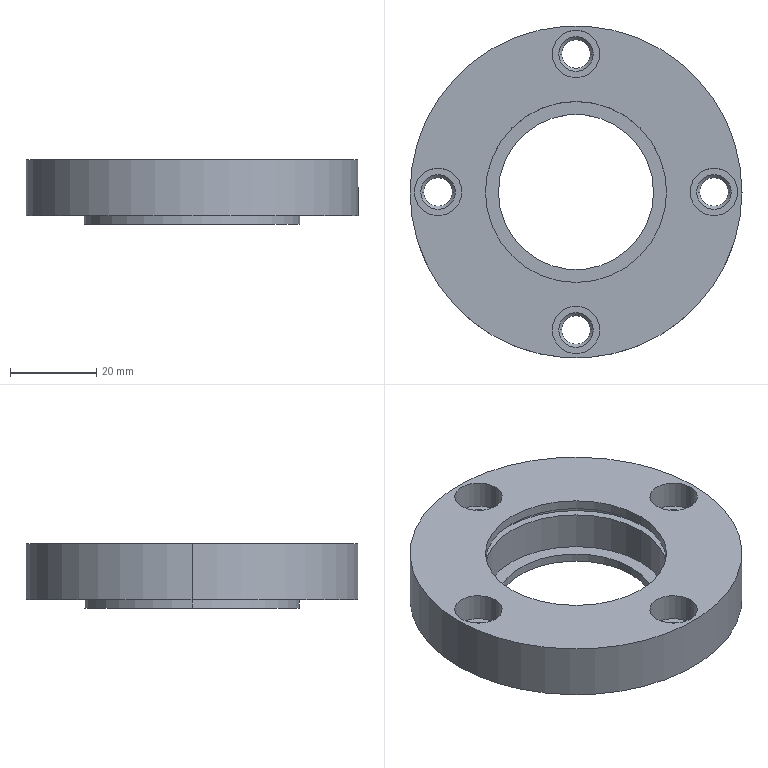Component | SolidWorks | BGRRB6905ZZ-1_housing_BGRRB6905ZZ-1 | 1 solid | 54 faces | box 77 x 77 x 15 mm | volume 40570 mm3 | cylinder 28 | cone 16 | plane 10 | commonest cylinder face diameters 11 x8 6.647 x8 42 x4 50 x2 45.5 x2 36 x2 77 x2 | material AISI 1045 Steel, cold drawn
build123d program:
from build123d import *

# Parameters (mm, degrees)
SKETCH1_R            = 38.5
BOSS_EXTRUDE1_DEPTH  = 15
LPATTERN1_COUNT      = 2
LPATTERN1_PITCH      = 45.255
LPATTERN1_COUNT_DIR2 = 2
LPATTERN1_PITCH_DIR2 = 45.255
SKETCH5_R            = 78
SKETCH5_R_2          = 25
CUT_EXTRUDE1_DEPTH   = 2


with BuildPart() as part:
    # Sketch1 → Boss-Extrude1 (new body)
    with BuildSketch(Plane(origin=(0, 0, 0), x_dir=(0, 0, -1), z_dir=(1, 0, 0))):
        Circle(SKETCH1_R)
    extrude(amount=BOSS_EXTRUDE1_DEPTH)

    # Sketch2 → Cut-Revolve1 (revolve, cut)
    with BuildSketch(Plane.XY, mode=Mode.PRIVATE) as cut_revolve1_sk:
        Polygon((0, 0), (0, 18), (2, 18), (2, 21), (11, 21), (11, 22.75), (12.8, 22.75), (12.8, 21), (15, 21), (15, 0), align=None)
    revolve(cut_revolve1_sk.sketch.rotate(Axis((15, 0, 0), (-1, 0, 0)), 270), axis=Axis((15, 0, 0), (-1, 0, 0)), mode=Mode.SUBTRACT)

    # Sketch3 → Cut-Revolve2 (revolve, cut)
    with BuildSketch(Plane.XY, mode=Mode.PRIVATE) as cut_revolve2_sk:
        Polygon((2, 32), (2, 36), (2.676, 35.324), (7.824, 35.324), (8.5, 36), (8.5, 37.5), (15, 37.5), (15, 32), align=None)
    cut_revolve2 = revolve(cut_revolve2_sk.sketch.rotate(Axis((15, 32, 0), (-1, 0, 0)), 270), axis=Axis((15, 32, 0), (-1, 0, 0)), mode=Mode.SUBTRACT)

    # LPattern1: Cut-Revolve2 2 × 2
    with Locations(*[Vector(0, -0.7071, 0.7071) * (i * LPATTERN1_PITCH) + Vector(0, -0.7071, -0.7071) * (j * LPATTERN1_PITCH_DIR2) for i in range(LPATTERN1_COUNT) for j in range(LPATTERN1_COUNT_DIR2) if (i, j) != (0, 0)]):
        add(cut_revolve2, mode=Mode.SUBTRACT)

    # Sketch5 → Cut-Extrude1 (cut)
    with BuildSketch(Plane(origin=(0, 0, 0), x_dir=(0, 0, -1), z_dir=(1, 0, 0))):
        Circle(SKETCH5_R)
        Circle(SKETCH5_R_2, mode=Mode.SUBTRACT)
    extrude(amount=CUT_EXTRUDE1_DEPTH, mode=Mode.SUBTRACT)


solid = part.part

# Placed as in the assembly
solid = solid.moved(Location((0, 0, 58), (0, -90, 0)))